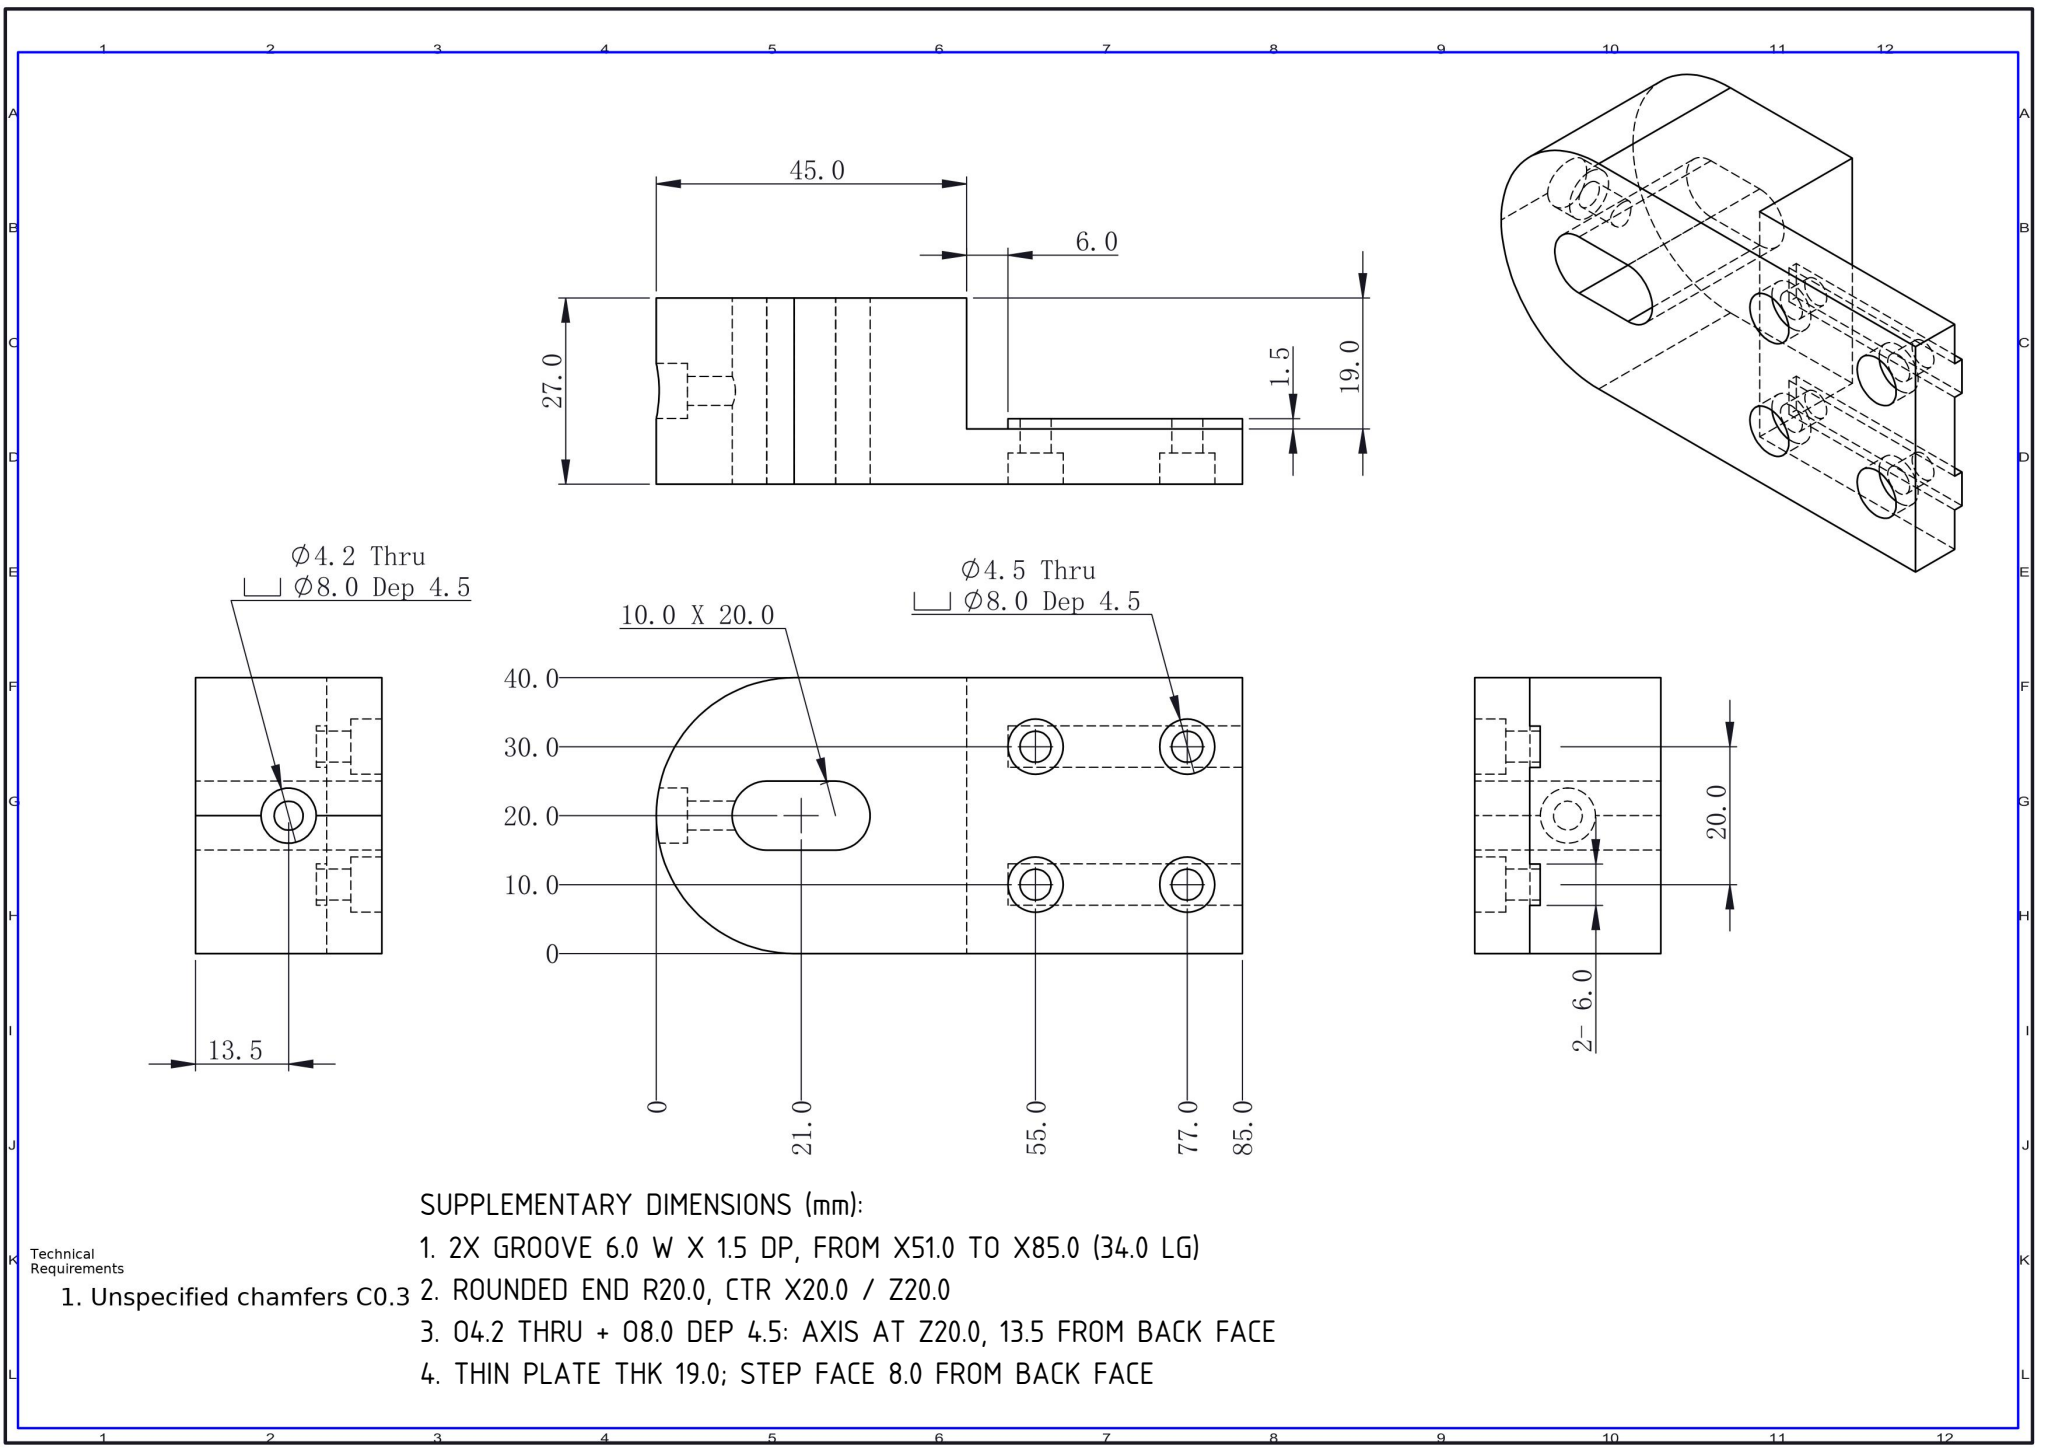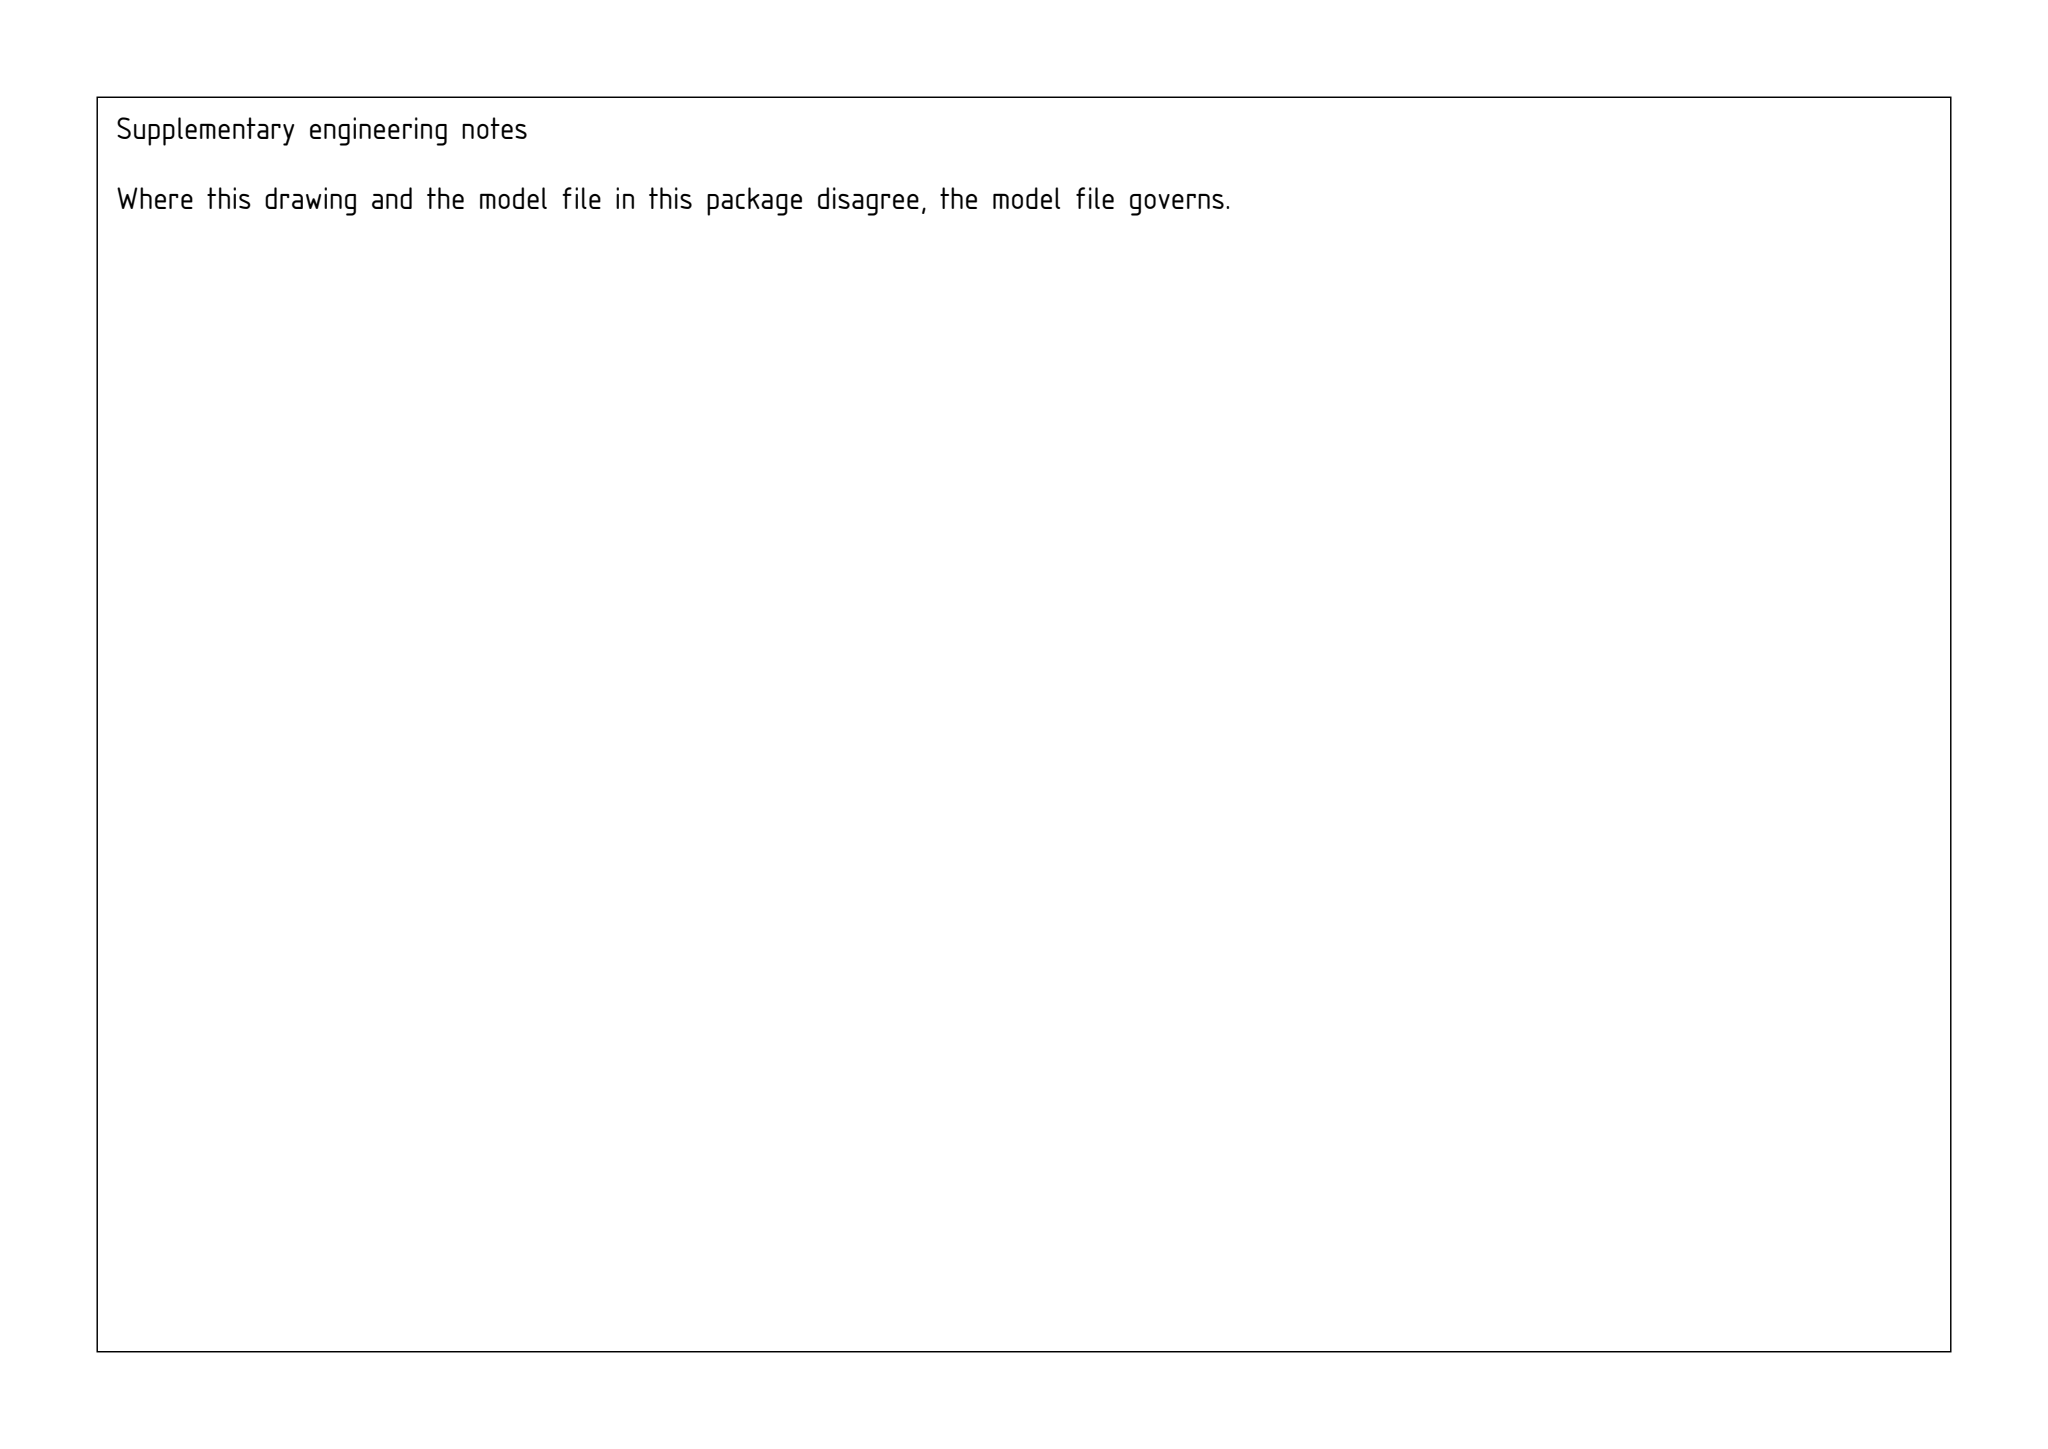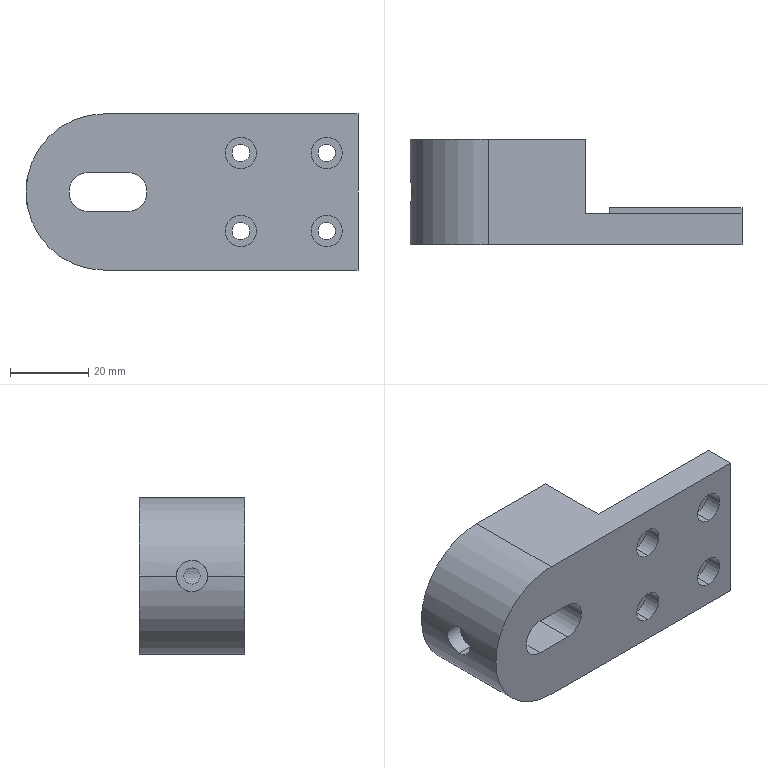Part | SolidWorks | mm | 1 solid | 46 faces | box 85 x 27 x 40 mm | volume 51020 mm3 | cylinder 24 | plane 22 | commonest cylinder face diameters 8 x10 4.5 x8 4.2 x2 10 x2 40 x2